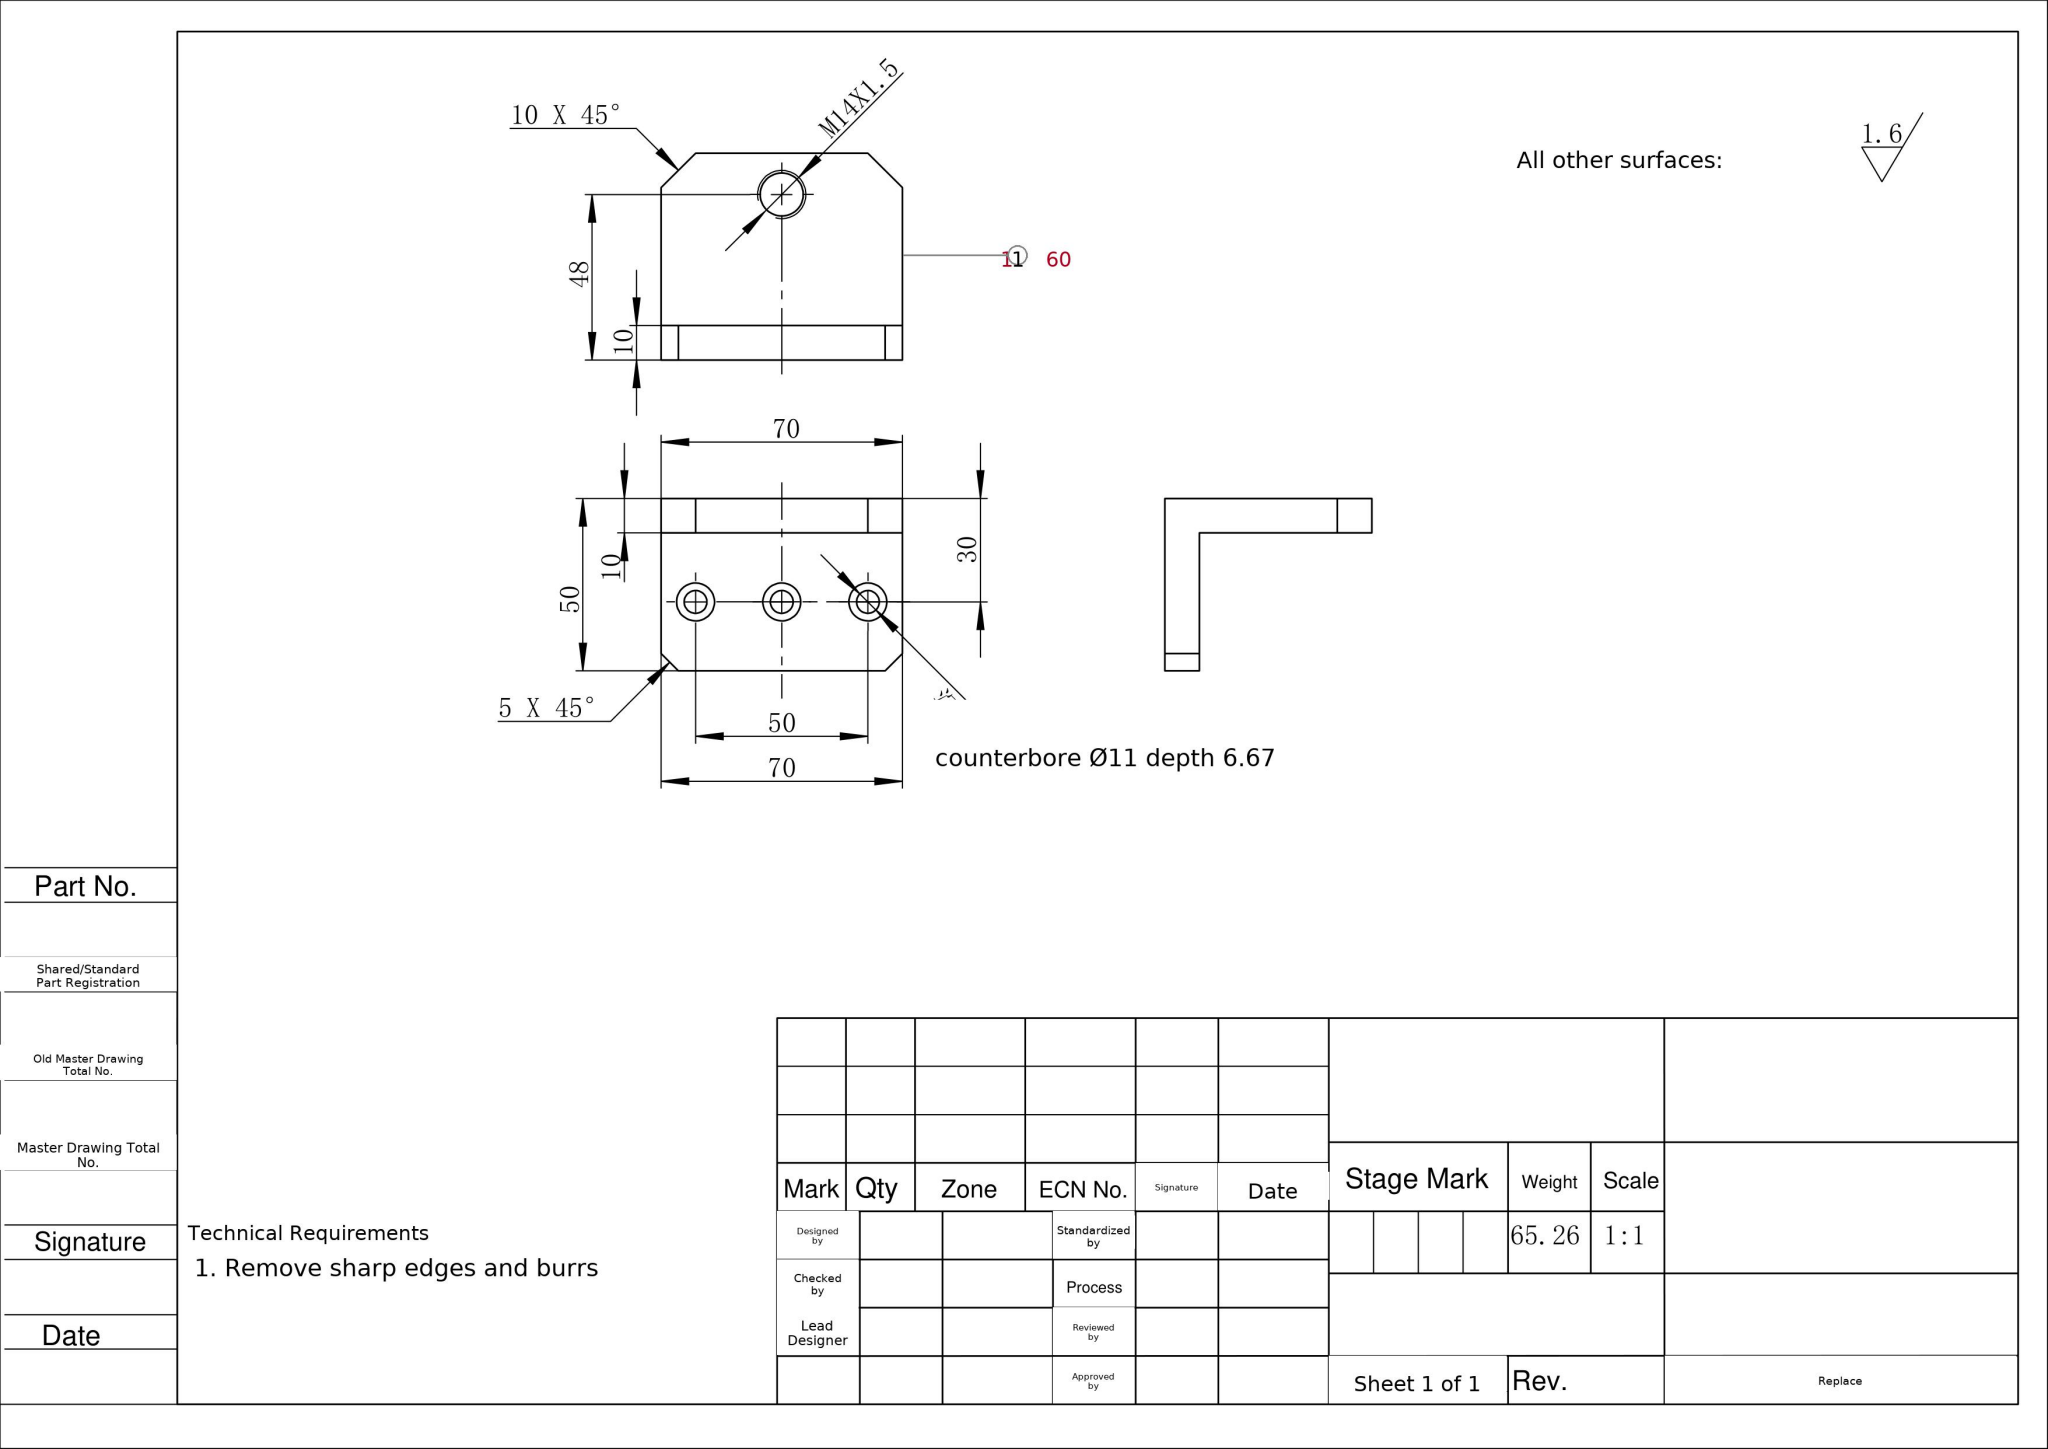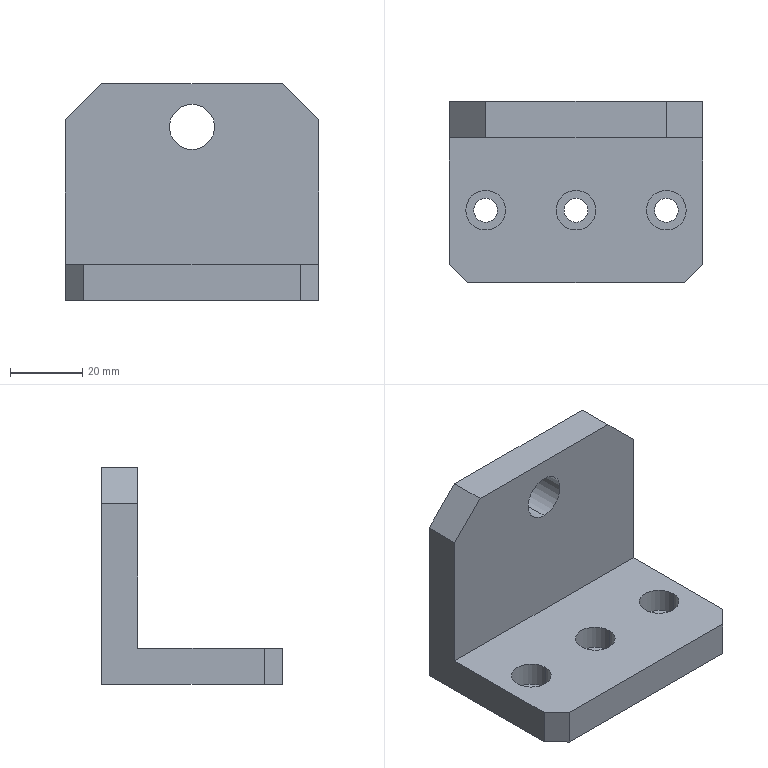Part | SolidWorks | mm | 1 solid | 29 faces | box 70 x 50 x 60 mm | volume 65256 mm3 | plane 15 | cylinder 14 | commonest cylinder face diameters 11 x6 6.6 x6 12.5 x2
build123d program:
from build123d import *

# Parameters (mm, degrees)
SKETCH1_W                                         = 70
SKETCH1_H                                         = 50
BOSS_EXTRUDE1_DEPTH                               = 10
SKETCH2_W                                         = 70
SKETCH2_H                                         = 10
BOSS_EXTRUDE2_DEPTH                               = 50
M14X1_5_TAPPED_HOLE1_D                            = 12.5
CHAMFER1_SIZE                                     = 10
CHAMFER2_SIZE                                     = 5
HOLE_SIZE_ACCORDING_TO_TYPE_1_OF_HEXA_D           = 6.6
HOLE_SIZE_ACCORDING_TO_TYPE_1_OF_HEXA_CBORE_D     = 11
HOLE_SIZE_ACCORDING_TO_TYPE_1_OF_HEXA_CBORE_DEPTH = 6.8


with BuildPart() as part:
    # Sketch1 → Boss-Extrude1 (new body)
    with BuildSketch(Plane.XY):
        with Locations((-1262.738, -1147.6)):
            Rectangle(SKETCH1_W, SKETCH1_H)
    extrude(amount=BOSS_EXTRUDE1_DEPTH)

    # Sketch2 → Boss-Extrude2 (add)
    with BuildSketch(Plane.XY.offset(10)):
        with Locations((-1262.738, -1127.6)):
            Rectangle(SKETCH2_W, SKETCH2_H)
    extrude(amount=BOSS_EXTRUDE2_DEPTH)

    # M14x1.5 Tapped Hole1 (through all)
    with Locations(Plane(origin=(0, -1132.6, 0), x_dir=(-1, 0, 0), z_dir=(0, -1, 0))):
        with Locations((1262.738, -48)):
            Hole(M14X1_5_TAPPED_HOLE1_D / 2)

    # Chamfer1
    chamfer1_edges = [part.edges().sort_by_distance(p)[0] for p in [
        (-1297.738, -1127.6, 60),
        (-1227.738, -1127.6, 60),
    ]]
    chamfer(chamfer1_edges, length=CHAMFER1_SIZE)

    # Chamfer2
    chamfer2_edges = [part.edges().sort_by_distance(p)[0] for p in [
        (-1227.738, -1172.6, 5),
        (-1297.738, -1172.6, 5),
    ]]
    chamfer(chamfer2_edges, length=CHAMFER2_SIZE)

    # Hole Size _ according to_ Type 1 of Hexa (through all)
    with Locations(Plane.XY.offset(10)):
        with Locations((-1287.738, -1152.6), (-1237.738, -1152.6), (-1262.738, -1152.6)):
            CounterBoreHole(HOLE_SIZE_ACCORDING_TO_TYPE_1_OF_HEXA_D / 2, HOLE_SIZE_ACCORDING_TO_TYPE_1_OF_HEXA_CBORE_D / 2, HOLE_SIZE_ACCORDING_TO_TYPE_1_OF_HEXA_CBORE_DEPTH)


solid = part.part
STEP:
#1=CARTESIAN_POINT('',(-1293.238,-1152.6,3.2));
#2=VERTEX_POINT('',#1);
#3=CARTESIAN_POINT('',(-1282.238,-1152.6,3.2));
#4=VERTEX_POINT('',#3);
#5=CARTESIAN_POINT('',(-1287.738,-1152.6,3.2));
#6=DIRECTION('',(0.,0.,1.));
#7=DIRECTION('',(1.,0.,0.));
#8=AXIS2_PLACEMENT_3D('',#5,#6,#7);
#9=CIRCLE('',#8,5.5);
#10=EDGE_CURVE('',#2,#4,#9,.T.);
#11=ORIENTED_EDGE('',*,*,#10,.F.);
#12=CARTESIAN_POINT('',(-1293.238,-1152.6,10.));
#13=VERTEX_POINT('',#12);
#14=CARTESIAN_POINT('',(-1293.238,-1152.6,10.));
#15=DIRECTION('',(0.,0.,1.));
#16=VECTOR('',#15,1000.);
#17=LINE('',#14,#16);
#18=EDGE_CURVE('',#2,#13,#17,.T.);
#19=ORIENTED_EDGE('',*,*,#18,.T.);
#20=CARTESIAN_POINT('',(-1282.238,-1152.6,10.));
#21=VERTEX_POINT('',#20);
#22=CARTESIAN_POINT('',(-1287.738,-1152.6,10.));
#23=DIRECTION('',(0.,0.,1.));
#24=DIRECTION('',(1.,0.,0.));
#25=AXIS2_PLACEMENT_3D('',#22,#23,#24);
#26=CIRCLE('',#25,5.5);
#27=EDGE_CURVE('',#13,#21,#26,.T.);
#28=ORIENTED_EDGE('',*,*,#27,.T.);
#29=CARTESIAN_POINT('',(-1282.238,-1152.6,10.));
#30=DIRECTION('',(0.,0.,1.));
#31=VECTOR('',#30,1000.);
#32=LINE('',#29,#31);
#33=EDGE_CURVE('',#4,#21,#32,.T.);
#34=ORIENTED_EDGE('',*,*,#33,.F.);
#35=EDGE_LOOP('',(#11,#19,#28,#34));
#36=FACE_OUTER_BOUND('',#35,.T.);
#37=CARTESIAN_POINT('',(-1287.738,-1152.6,10.));
#38=DIRECTION('',(0.,0.,1.));
#39=DIRECTION('',(1.,0.,0.));
#40=AXIS2_PLACEMENT_3D('',#37,#38,#39);
#41=CYLINDRICAL_SURFACE('',#40,5.5);
#42=ADVANCED_FACE('',(#36),#41,.F.);
#43=CARTESIAN_POINT('',(-1291.038,-1152.6,0.));
#44=VERTEX_POINT('',#43);
#45=CARTESIAN_POINT('',(-1284.438,-1152.6,0.));
#46=VERTEX_POINT('',#45);
#47=CARTESIAN_POINT('',(-1287.738,-1152.6,0.));
#48=DIRECTION('',(0.,0.,1.));
#49=DIRECTION('',(1.,0.,0.));
#50=AXIS2_PLACEMENT_3D('',#47,#48,#49);
#51=CIRCLE('',#50,3.3);
#52=EDGE_CURVE('',#44,#46,#51,.T.);
#53=ORIENTED_EDGE('',*,*,#52,.F.);
#54=CARTESIAN_POINT('',(-1291.038,-1152.6,3.2));
#55=VERTEX_POINT('',#54);
#56=CARTESIAN_POINT('',(-1291.038,-1152.6,10.));
#57=DIRECTION('',(0.,0.,1.));
#58=VECTOR('',#57,1000.);
#59=LINE('',#56,#58);
#60=EDGE_CURVE('',#44,#55,#59,.T.);
#61=ORIENTED_EDGE('',*,*,#60,.T.);
#62=CARTESIAN_POINT('',(-1284.438,-1152.6,3.2));
#63=VERTEX_POINT('',#62);
#64=CARTESIAN_POINT('',(-1287.738,-1152.6,3.2));
#65=DIRECTION('',(0.,0.,1.));
#66=DIRECTION('',(1.,0.,0.));
#67=AXIS2_PLACEMENT_3D('',#64,#65,#66);
#68=CIRCLE('',#67,3.3);
#69=EDGE_CURVE('',#55,#63,#68,.T.);
#70=ORIENTED_EDGE('',*,*,#69,.T.);
#71=CARTESIAN_POINT('',(-1284.438,-1152.6,10.));
#72=DIRECTION('',(0.,0.,1.));
#73=VECTOR('',#72,1000.);
#74=LINE('',#71,#73);
#75=EDGE_CURVE('',#46,#63,#74,.T.);
#76=ORIENTED_EDGE('',*,*,#75,.F.);
#77=EDGE_LOOP('',(#53,#61,#70,#76));
#78=FACE_OUTER_BOUND('',#77,.T.);
#79=CARTESIAN_POINT('',(-1287.738,-1152.6,10.));
#80=DIRECTION('',(0.,0.,1.));
#81=DIRECTION('',(1.,0.,0.));
#82=AXIS2_PLACEMENT_3D('',#79,#80,#81);
#83=CYLINDRICAL_SURFACE('',#82,3.3);
#84=ADVANCED_FACE('',(#78),#83,.F.);
#85=CARTESIAN_POINT('',(-1243.238,-1152.6,3.2));
#86=VERTEX_POINT('',#85);
#87=CARTESIAN_POINT('',(-1232.238,-1152.6,3.2));
#88=VERTEX_POINT('',#87);
#89=CARTESIAN_POINT('',(-1237.738,-1152.6,3.2));
#90=DIRECTION('',(0.,0.,1.));
#91=DIRECTION('',(1.,0.,0.));
#92=AXIS2_PLACEMENT_3D('',#89,#90,#91);
#93=CIRCLE('',#92,5.5);
#94=EDGE_CURVE('',#86,#88,#93,.T.);
#95=ORIENTED_EDGE('',*,*,#94,.F.);
#96=CARTESIAN_POINT('',(-1243.238,-1152.6,10.));
#97=VERTEX_POINT('',#96);
#98=CARTESIAN_POINT('',(-1243.238,-1152.6,10.));
#99=DIRECTION('',(0.,0.,1.));
#100=VECTOR('',#99,1000.);
#101=LINE('',#98,#100);
#102=EDGE_CURVE('',#86,#97,#101,.T.);
#103=ORIENTED_EDGE('',*,*,#102,.T.);
#104=CARTESIAN_POINT('',(-1232.238,-1152.6,10.));
#105=VERTEX_POINT('',#104);
#106=CARTESIAN_POINT('',(-1237.738,-1152.6,10.));
#107=DIRECTION('',(0.,0.,1.));
#108=DIRECTION('',(1.,0.,0.));
#109=AXIS2_PLACEMENT_3D('',#106,#107,#108);
#110=CIRCLE('',#109,5.5);
#111=EDGE_CURVE('',#97,#105,#110,.T.);
#112=ORIENTED_EDGE('',*,*,#111,.T.);
#113=CARTESIAN_POINT('',(-1232.238,-1152.6,10.));
#114=DIRECTION('',(0.,0.,1.));
#115=VECTOR('',#114,1000.);
#116=LINE('',#113,#115);
#117=EDGE_CURVE('',#88,#105,#116,.T.);
#118=ORIENTED_EDGE('',*,*,#117,.F.);
#119=EDGE_LOOP('',(#95,#103,#112,#118));
#120=FACE_OUTER_BOUND('',#119,.T.);
#121=CARTESIAN_POINT('',(-1237.738,-1152.6,10.));
#122=DIRECTION('',(0.,0.,1.));
#123=DIRECTION('',(1.,0.,0.));
#124=AXIS2_PLACEMENT_3D('',#121,#122,#123);
#125=CYLINDRICAL_SURFACE('',#124,5.5);
#126=ADVANCED_FACE('',(#120),#125,.F.);
#127=CARTESIAN_POINT('',(-1241.038,-1152.6,0.));
#128=VERTEX_POINT('',#127);
#129=CARTESIAN_POINT('',(-1234.438,-1152.6,0.));
#130=VERTEX_POINT('',#129);
#131=CARTESIAN_POINT('',(-1237.738,-1152.6,0.));
#132=DIRECTION('',(0.,0.,1.));
#133=DIRECTION('',(1.,0.,0.));
#134=AXIS2_PLACEMENT_3D('',#131,#132,#133);
#135=CIRCLE('',#134,3.3);
#136=EDGE_CURVE('',#128,#130,#135,.T.);
#137=ORIENTED_EDGE('',*,*,#136,.F.);
#138=CARTESIAN_POINT('',(-1241.038,-1152.6,3.2));
#139=VERTEX_POINT('',#138);
#140=CARTESIAN_POINT('',(-1241.038,-1152.6,10.));
#141=DIRECTION('',(0.,0.,1.));
#142=VECTOR('',#141,1000.);
#143=LINE('',#140,#142);
#144=EDGE_CURVE('',#128,#139,#143,.T.);
#145=ORIENTED_EDGE('',*,*,#144,.T.);
#146=CARTESIAN_POINT('',(-1234.438,-1152.6,3.2));
#147=VERTEX_POINT('',#146);
#148=CARTESIAN_POINT('',(-1237.738,-1152.6,3.2));
#149=DIRECTION('',(0.,0.,1.));
#150=DIRECTION('',(1.,0.,0.));
#151=AXIS2_PLACEMENT_3D('',#148,#149,#150);
#152=CIRCLE('',#151,3.3);
#153=EDGE_CURVE('',#139,#147,#152,.T.);
#154=ORIENTED_EDGE('',*,*,#153,.T.);
#155=CARTESIAN_POINT('',(-1234.438,-1152.6,10.));
#156=DIRECTION('',(0.,0.,1.));
#157=VECTOR('',#156,1000.);
#158=LINE('',#155,#157);
#159=EDGE_CURVE('',#130,#147,#158,.T.);
#160=ORIENTED_EDGE('',*,*,#159,.F.);
#161=EDGE_LOOP('',(#137,#145,#154,#160));
#162=FACE_OUTER_BOUND('',#161,.T.);
#163=CARTESIAN_POINT('',(-1237.738,-1152.6,10.));
#164=DIRECTION('',(0.,0.,1.));
#165=DIRECTION('',(1.,0.,0.));
#166=AXIS2_PLACEMENT_3D('',#163,#164,#165);
#167=CYLINDRICAL_SURFACE('',#166,3.3);
#168=ADVANCED_FACE('',(#162),#167,.F.);
#169=CARTESIAN_POINT('',(-1268.238,-1152.6,3.2));
#170=VERTEX_POINT('',#169);
#171=CARTESIAN_POINT('',(-1257.238,-1152.6,3.2));
#172=VERTEX_POINT('',#171);
#173=CARTESIAN_POINT('',(-1262.738,-1152.6,3.2));
#174=DIRECTION('',(0.,0.,1.));
#175=DIRECTION('',(1.,0.,0.));
#176=AXIS2_PLACEMENT_3D('',#173,#174,#175);
#177=CIRCLE('',#176,5.5);
#178=EDGE_CURVE('',#170,#172,#177,.T.);
#179=ORIENTED_EDGE('',*,*,#178,.F.);
#180=CARTESIAN_POINT('',(-1268.238,-1152.6,10.));
#181=VERTEX_POINT('',#180);
#182=CARTESIAN_POINT('',(-1268.238,-1152.6,10.));
#183=DIRECTION('',(0.,0.,1.));
#184=VECTOR('',#183,1000.);
#185=LINE('',#182,#184);
#186=EDGE_CURVE('',#170,#181,#185,.T.);
#187=ORIENTED_EDGE('',*,*,#186,.T.);
#188=CARTESIAN_POINT('',(-1257.238,-1152.6,10.));
#189=VERTEX_POINT('',#188);
#190=CARTESIAN_POINT('',(-1262.738,-1152.6,10.));
#191=DIRECTION('',(0.,0.,1.));
#192=DIRECTION('',(1.,0.,0.));
#193=AXIS2_PLACEMENT_3D('',#190,#191,#192);
#194=CIRCLE('',#193,5.5);
#195=EDGE_CURVE('',#181,#189,#194,.T.);
#196=ORIENTED_EDGE('',*,*,#195,.T.);
#197=CARTESIAN_POINT('',(-1257.238,-1152.6,10.));
#198=DIRECTION('',(0.,0.,1.));
#199=VECTOR('',#198,1000.);
#200=LINE('',#197,#199);
#201=EDGE_CURVE('',#172,#189,#200,.T.);
#202=ORIENTED_EDGE('',*,*,#201,.F.);
#203=EDGE_LOOP('',(#179,#187,#196,#202));
#204=FACE_OUTER_BOUND('',#203,.T.);
#205=CARTESIAN_POINT('',(-1262.738,-1152.6,10.));
#206=DIRECTION('',(0.,0.,1.));
#207=DIRECTION('',(1.,0.,0.));
#208=AXIS2_PLACEMENT_3D('',#205,#206,#207);
#209=CYLINDRICAL_SURFACE('',#208,5.5);
#210=ADVANCED_FACE('',(#204),#209,.F.);
#211=CARTESIAN_POINT('',(-1266.038,-1152.6,0.));
#212=VERTEX_POINT('',#211);
#213=CARTESIAN_POINT('',(-1259.438,-1152.6,0.));
#214=VERTEX_POINT('',#213);
#215=CARTESIAN_POINT('',(-1262.738,-1152.6,0.));
#216=DIRECTION('',(0.,0.,1.));
#217=DIRECTION('',(1.,0.,0.));
#218=AXIS2_PLACEMENT_3D('',#215,#216,#217);
#219=CIRCLE('',#218,3.3);
#220=EDGE_CURVE('',#212,#214,#219,.T.);
#221=ORIENTED_EDGE('',*,*,#220,.F.);
#222=CARTESIAN_POINT('',(-1266.038,-1152.6,3.2));
#223=VERTEX_POINT('',#222);
#224=CARTESIAN_POINT('',(-1266.038,-1152.6,10.));
#225=DIRECTION('',(0.,0.,1.));
#226=VECTOR('',#225,1000.);
#227=LINE('',#224,#226);
#228=EDGE_CURVE('',#212,#223,#227,.T.);
#229=ORIENTED_EDGE('',*,*,#228,.T.);
#230=CARTESIAN_POINT('',(-1259.438,-1152.6,3.2));
#231=VERTEX_POINT('',#230);
#232=CARTESIAN_POINT('',(-1262.738,-1152.6,3.2));
#233=DIRECTION('',(0.,0.,1.));
#234=DIRECTION('',(1.,0.,0.));
#235=AXIS2_PLACEMENT_3D('',#232,#233,#234);
#236=CIRCLE('',#235,3.3);
#237=EDGE_CURVE('',#223,#231,#236,.T.);
#238=ORIENTED_EDGE('',*,*,#237,.T.);
#239=CARTESIAN_POINT('',(-1259.438,-1152.6,10.));
#240=DIRECTION('',(0.,0.,1.));
#241=VECTOR('',#240,1000.);
#242=LINE('',#239,#241);
#243=EDGE_CURVE('',#214,#231,#242,.T.);
#244=ORIENTED_EDGE('',*,*,#243,.F.);
#245=EDGE_LOOP('',(#221,#229,#238,#244));
#246=FACE_OUTER_BOUND('',#245,.T.);
#247=CARTESIAN_POINT('',(-1262.738,-1152.6,10.));
#248=DIRECTION('',(0.,0.,1.));
#249=DIRECTION('',(1.,0.,0.));
#250=AXIS2_PLACEMENT_3D('',#247,#248,#249);
#251=CYLINDRICAL_SURFACE('',#250,3.3);
#252=ADVANCED_FACE('',(#246),#251,.F.);
#253=CARTESIAN_POINT('',(-1262.738,-1122.6,54.25));
#254=VERTEX_POINT('',#253);
#255=CARTESIAN_POINT('',(-1262.738,-1122.6,41.75));
#256=VERTEX_POINT('',#255);
#257=CARTESIAN_POINT('',(-1262.738,-1122.6,48.));
#258=DIRECTION('',(0.,-1.,0.));
#259=DIRECTION('',(0.,0.,-1.));
#260=AXIS2_PLACEMENT_3D('',#257,#258,#259);
#261=CIRCLE('',#260,6.25);
#262=EDGE_CURVE('',#254,#256,#261,.T.);
#263=ORIENTED_EDGE('',*,*,#262,.F.);
#264=CARTESIAN_POINT('',(-1262.738,-1132.6,54.25));
#265=VERTEX_POINT('',#264);
#266=CARTESIAN_POINT('',(-1262.738,-1132.6,54.25));
#267=DIRECTION('',(0.,-1.,0.));
#268=VECTOR('',#267,1000.);
#269=LINE('',#266,#268);
#270=EDGE_CURVE('',#254,#265,#269,.T.);
#271=ORIENTED_EDGE('',*,*,#270,.T.);
#272=CARTESIAN_POINT('',(-1262.738,-1132.6,41.75));
#273=VERTEX_POINT('',#272);
#274=CARTESIAN_POINT('',(-1262.738,-1132.6,48.));
#275=DIRECTION('',(0.,-1.,0.));
#276=DIRECTION('',(0.,0.,-1.));
#277=AXIS2_PLACEMENT_3D('',#274,#275,#276);
#278=CIRCLE('',#277,6.25);
#279=EDGE_CURVE('',#265,#273,#278,.T.);
#280=ORIENTED_EDGE('',*,*,#279,.T.);
#281=CARTESIAN_POINT('',(-1262.738,-1132.6,41.75));
#282=DIRECTION('',(0.,-1.,0.));
#283=VECTOR('',#282,1000.);
#284=LINE('',#281,#283);
#285=EDGE_CURVE('',#256,#273,#284,.T.);
#286=ORIENTED_EDGE('',*,*,#285,.F.);
#287=EDGE_LOOP('',(#263,#271,#280,#286));
#288=FACE_OUTER_BOUND('',#287,.T.);
#289=CARTESIAN_POINT('',(-1262.738,-1132.6,48.));
#290=DIRECTION('',(0.,-1.,0.));
#291=DIRECTION('',(0.,0.,-1.));
#292=AXIS2_PLACEMENT_3D('',#289,#290,#291);
#293=CYLINDRICAL_SURFACE('',#292,6.25);
#294=ADVANCED_FACE('',(#288),#293,.F.);
#295=CARTESIAN_POINT('',(-1297.738,-1122.6,0.));
#296=VERTEX_POINT('',#295);
#297=CARTESIAN_POINT('',(-1297.738,-1167.6,0.));
#298=VERTEX_POINT('',#297);
#299=CARTESIAN_POINT('',(-1297.738,-1122.6,0.));
#300=DIRECTION('',(0.,-1.,0.));
#301=VECTOR('',#300,1000.);
#302=LINE('',#299,#301);
#303=EDGE_CURVE('',#296,#298,#302,.T.);
#304=ORIENTED_EDGE('',*,*,#303,.T.);
#305=CARTESIAN_POINT('',(-1297.738,-1167.6,10.));
#306=VERTEX_POINT('',#305);
#307=CARTESIAN_POINT('',(-1297.738,-1167.6,10.));
#308=DIRECTION('',(0.,0.,1.));
#309=VECTOR('',#308,1000.);
#310=LINE('',#307,#309);
#311=EDGE_CURVE('',#298,#306,#310,.T.);
#312=ORIENTED_EDGE('',*,*,#311,.T.);
#313=CARTESIAN_POINT('',(-1297.738,-1132.6,10.));
#314=VERTEX_POINT('',#313);
#315=CARTESIAN_POINT('',(-1297.738,-1122.6,10.));
#316=DIRECTION('',(0.,-1.,0.));
#317=VECTOR('',#316,1000.);
#318=LINE('',#315,#317);
#319=EDGE_CURVE('',#314,#306,#318,.T.);
#320=ORIENTED_EDGE('',*,*,#319,.F.);
#321=CARTESIAN_POINT('',(-1297.738,-1132.6,50.));
#322=VERTEX_POINT('',#321);
#323=CARTESIAN_POINT('',(-1297.738,-1132.6,60.));
#324=DIRECTION('',(0.,0.,-1.));
#325=VECTOR('',#324,1000.);
#326=LINE('',#323,#325);
#327=EDGE_CURVE('',#322,#314,#326,.T.);
#328=ORIENTED_EDGE('',*,*,#327,.F.);
#329=CARTESIAN_POINT('',(-1297.738,-1122.6,50.));
#330=VERTEX_POINT('',#329);
#331=CARTESIAN_POINT('',(-1297.738,-1122.6,50.));
#332=DIRECTION('',(-0.,1.,0.));
#333=VECTOR('',#332,1000.);
#334=LINE('',#331,#333);
#335=EDGE_CURVE('',#322,#330,#334,.T.);
#336=ORIENTED_EDGE('',*,*,#335,.T.);
#337=CARTESIAN_POINT('',(-1297.738,-1122.6,10.));
#338=DIRECTION('',(0.,0.,-1.));
#339=VECTOR('',#338,1000.);
#340=LINE('',#337,#339);
#341=EDGE_CURVE('',#330,#296,#340,.T.);
#342=ORIENTED_EDGE('',*,*,#341,.T.);
#343=EDGE_LOOP('',(#304,#312,#320,#328,#336,#342));
#344=FACE_OUTER_BOUND('',#343,.T.);
#345=CARTESIAN_POINT('',(-1297.738,-1122.6,10.));
#346=DIRECTION('',(1.,0.,0.));
#347=DIRECTION('',(-0.,1.,0.));
#348=AXIS2_PLACEMENT_3D('',#345,#346,#347);
#349=PLANE('',#348);
#350=ADVANCED_FACE('',(#344),#349,.F.);
#351=CARTESIAN_POINT('',(-1292.738,-1172.6,0.));
#352=VERTEX_POINT('',#351);
#353=CARTESIAN_POINT('',(-1232.738,-1172.6,0.));
#354=VERTEX_POINT('',#353);
#355=CARTESIAN_POINT('',(-1297.738,-1172.6,0.));
#356=DIRECTION('',(1.,0.,0.));
#357=VECTOR('',#356,1000.);
#358=LINE('',#355,#357);
#359=EDGE_CURVE('',#352,#354,#358,.T.);
#360=ORIENTED_EDGE('',*,*,#359,.T.);
#361=CARTESIAN_POINT('',(-1232.738,-1172.6,10.));
#362=VERTEX_POINT('',#361);
#363=CARTESIAN_POINT('',(-1232.738,-1172.6,10.));
#364=DIRECTION('',(0.,0.,1.));
#365=VECTOR('',#364,1000.);
#366=LINE('',#363,#365);
#367=EDGE_CURVE('',#354,#362,#366,.T.);
#368=ORIENTED_EDGE('',*,*,#367,.T.);
#369=CARTESIAN_POINT('',(-1292.738,-1172.6,10.));
#370=VERTEX_POINT('',#369);
#371=CARTESIAN_POINT('',(-1297.738,-1172.6,10.));
#372=DIRECTION('',(1.,0.,0.));
#373=VECTOR('',#372,1000.);
#374=LINE('',#371,#373);
#375=EDGE_CURVE('',#370,#362,#374,.T.);
#376=ORIENTED_EDGE('',*,*,#375,.F.);
#377=CARTESIAN_POINT('',(-1292.738,-1172.6,10.));
#378=DIRECTION('',(0.,0.,-1.));
#379=VECTOR('',#378,1000.);
#380=LINE('',#377,#379);
#381=EDGE_CURVE('',#370,#352,#380,.T.);
#382=ORIENTED_EDGE('',*,*,#381,.T.);
#383=EDGE_LOOP('',(#360,#368,#376,#382));
#384=FACE_OUTER_BOUND('',#383,.T.);
#385=CARTESIAN_POINT('',(-1297.738,-1172.6,10.));
#386=DIRECTION('',(0.,1.,0.));
#387=DIRECTION('',(0.,0.,1.));
#388=AXIS2_PLACEMENT_3D('',#385,#386,#387);
#389=PLANE('',#388);
#390=ADVANCED_FACE('',(#384),#389,.F.);
#391=CARTESIAN_POINT('',(-1227.738,-1167.6,10.));
#392=VERTEX_POINT('',#391);
#393=CARTESIAN_POINT('',(-1227.738,-1132.6,10.));
#394=VERTEX_POINT('',#393);
#395=CARTESIAN_POINT('',(-1227.738,-1122.6,10.));
#396=DIRECTION('',(0.,1.,0.));
#397=VECTOR('',#396,1000.);
#398=LINE('',#395,#397);
#399=EDGE_CURVE('',#392,#394,#398,.T.);
#400=ORIENTED_EDGE('',*,*,#399,.F.);
#401=CARTESIAN_POINT('',(-1227.738,-1167.6,0.));
#402=VERTEX_POINT('',#401);
#403=CARTESIAN_POINT('',(-1227.738,-1167.6,10.));
#404=DIRECTION('',(0.,0.,-1.));
#405=VECTOR('',#404,1000.);
#406=LINE('',#403,#405);
#407=EDGE_CURVE('',#392,#402,#406,.T.);
#408=ORIENTED_EDGE('',*,*,#407,.T.);
#409=CARTESIAN_POINT('',(-1227.738,-1122.6,0.));
#410=VERTEX_POINT('',#409);
#411=CARTESIAN_POINT('',(-1227.738,-1122.6,0.));
#412=DIRECTION('',(0.,1.,0.));
#413=VECTOR('',#412,1000.);
#414=LINE('',#411,#413);
#415=EDGE_CURVE('',#402,#410,#414,.T.);
#416=ORIENTED_EDGE('',*,*,#415,.T.);
#417=CARTESIAN_POINT('',(-1227.738,-1122.6,50.));
#418=VERTEX_POINT('',#417);
#419=CARTESIAN_POINT('',(-1227.738,-1122.6,10.));
#420=DIRECTION('',(0.,0.,-1.));
#421=VECTOR('',#420,1000.);
#422=LINE('',#419,#421);
#423=EDGE_CURVE('',#418,#410,#422,.T.);
#424=ORIENTED_EDGE('',*,*,#423,.F.);
#425=CARTESIAN_POINT('',(-1227.738,-1132.6,50.));
#426=VERTEX_POINT('',#425);
#427=CARTESIAN_POINT('',(-1227.738,-1132.6,50.));
#428=DIRECTION('',(-0.,-1.,0.));
#429=VECTOR('',#428,1000.);
#430=LINE('',#427,#429);
#431=EDGE_CURVE('',#418,#426,#430,.T.);
#432=ORIENTED_EDGE('',*,*,#431,.T.);
#433=CARTESIAN_POINT('',(-1227.738,-1132.6,60.));
#434=DIRECTION('',(0.,0.,-1.));
#435=VECTOR('',#434,1000.);
#436=LINE('',#433,#435);
#437=EDGE_CURVE('',#426,#394,#436,.T.);
#438=ORIENTED_EDGE('',*,*,#437,.T.);
#439=EDGE_LOOP('',(#400,#408,#416,#424,#432,#438));
#440=FACE_OUTER_BOUND('',#439,.T.);
#441=CARTESIAN_POINT('',(-1227.738,-1122.6,10.));
#442=DIRECTION('',(-1.,0.,0.));
#443=DIRECTION('',(-0.,-1.,0.));
#444=AXIS2_PLACEMENT_3D('',#441,#442,#443);
#445=PLANE('',#444);
#446=ADVANCED_FACE('',(#440),#445,.F.);
#447=CARTESIAN_POINT('',(-1262.738,-1122.6,48.));
#448=DIRECTION('',(0.,-1.,0.));
#449=DIRECTION('',(0.,0.,-1.));
#450=AXIS2_PLACEMENT_3D('',#447,#448,#449);
#451=CIRCLE('',#450,6.25);
#452=EDGE_CURVE('',#256,#254,#451,.T.);
#453=ORIENTED_EDGE('',*,*,#452,.T.);
#454=ORIENTED_EDGE('',*,*,#262,.T.);
#455=EDGE_LOOP('',(#453,#454));
#456=FACE_BOUND('',#455,.T.);
#457=CARTESIAN_POINT('',(-1237.738,-1122.6,60.));
#458=VERTEX_POINT('',#457);
#459=CARTESIAN_POINT('',(-1287.738,-1122.6,60.));
#460=VERTEX_POINT('',#459);
#461=CARTESIAN_POINT('',(-1297.738,-1122.6,60.));
#462=DIRECTION('',(-1.,0.,0.));
#463=VECTOR('',#462,1000.);
#464=LINE('',#461,#463);
#465=EDGE_CURVE('',#458,#460,#464,.T.);
#466=ORIENTED_EDGE('',*,*,#465,.F.);
#467=CARTESIAN_POINT('',(-1237.738,-1122.6,60.));
#468=DIRECTION('',(0.7071,0.,-0.7071));
#469=VECTOR('',#468,1000.);
#470=LINE('',#467,#469);
#471=EDGE_CURVE('',#458,#418,#470,.T.);
#472=ORIENTED_EDGE('',*,*,#471,.T.);
#473=ORIENTED_EDGE('',*,*,#423,.T.);
#474=CARTESIAN_POINT('',(-1297.738,-1122.6,0.));
#475=DIRECTION('',(-1.,0.,0.));
#476=VECTOR('',#475,1000.);
#477=LINE('',#474,#476);
#478=EDGE_CURVE('',#410,#296,#477,.T.);
#479=ORIENTED_EDGE('',*,*,#478,.T.);
#480=ORIENTED_EDGE('',*,*,#341,.F.);
#481=CARTESIAN_POINT('',(-1287.738,-1122.6,60.));
#482=DIRECTION('',(0.7071,0.,0.7071));
#483=VECTOR('',#482,1000.);
#484=LINE('',#481,#483);
#485=EDGE_CURVE('',#330,#460,#484,.T.);
#486=ORIENTED_EDGE('',*,*,#485,.T.);
#487=EDGE_LOOP('',(#466,#472,#473,#479,#480,#486));
#488=FACE_OUTER_BOUND('',#487,.T.);
#489=CARTESIAN_POINT('',(-1297.738,-1122.6,10.));
#490=DIRECTION('',(0.,-1.,0.));
#491=DIRECTION('',(0.,0.,-1.));
#492=AXIS2_PLACEMENT_3D('',#489,#490,#491);
#493=PLANE('',#492);
#494=ADVANCED_FACE('',(#456,#488),#493,.F.);
#495=CARTESIAN_POINT('',(-1287.738,-1152.6,10.));
#496=DIRECTION('',(0.,0.,1.));
#497=DIRECTION('',(1.,0.,0.));
#498=AXIS2_PLACEMENT_3D('',#495,#496,#497);
#499=CIRCLE('',#498,5.5);
#500=EDGE_CURVE('',#21,#13,#499,.T.);
#501=ORIENTED_EDGE('',*,*,#500,.F.);
#502=ORIENTED_EDGE('',*,*,#27,.F.);
#503=EDGE_LOOP('',(#501,#502));
#504=FACE_BOUND('',#503,.T.);
#505=CARTESIAN_POINT('',(-1237.738,-1152.6,10.));
#506=DIRECTION('',(0.,0.,1.));
#507=DIRECTION('',(1.,0.,0.));
#508=AXIS2_PLACEMENT_3D('',#505,#506,#507);
#509=CIRCLE('',#508,5.5);
#510=EDGE_CURVE('',#105,#97,#509,.T.);
#511=ORIENTED_EDGE('',*,*,#510,.F.);
#512=ORIENTED_EDGE('',*,*,#111,.F.);
#513=EDGE_LOOP('',(#511,#512));
#514=FACE_BOUND('',#513,.T.);
#515=CARTESIAN_POINT('',(-1262.738,-1152.6,10.));
#516=DIRECTION('',(0.,0.,1.));
#517=DIRECTION('',(1.,0.,0.));
#518=AXIS2_PLACEMENT_3D('',#515,#516,#517);
#519=CIRCLE('',#518,5.5);
#520=EDGE_CURVE('',#189,#181,#519,.T.);
#521=ORIENTED_EDGE('',*,*,#520,.F.);
#522=ORIENTED_EDGE('',*,*,#195,.F.);
#523=EDGE_LOOP('',(#521,#522));
#524=FACE_BOUND('',#523,.T.);
#525=ORIENTED_EDGE('',*,*,#375,.T.);
#526=CARTESIAN_POINT('',(-30.069,30.069,10.));
#527=DIRECTION('',(0.7071,0.7071,0.));
#528=VECTOR('',#527,1000.);
#529=LINE('',#526,#528);
#530=EDGE_CURVE('',#362,#392,#529,.T.);
#531=ORIENTED_EDGE('',*,*,#530,.T.);
#532=ORIENTED_EDGE('',*,*,#399,.T.);
#533=CARTESIAN_POINT('',(-1297.738,-1132.6,10.));
#534=DIRECTION('',(1.,0.,0.));
#535=VECTOR('',#534,1000.);
#536=LINE('',#533,#535);
#537=EDGE_CURVE('',#314,#394,#536,.T.);
#538=ORIENTED_EDGE('',*,*,#537,.F.);
#539=ORIENTED_EDGE('',*,*,#319,.T.);
#540=CARTESIAN_POINT('',(-1232.669,-1232.669,10.));
#541=DIRECTION('',(0.7071,-0.7071,0.));
#542=VECTOR('',#541,1000.);
#543=LINE('',#540,#542);
#544=EDGE_CURVE('',#306,#370,#543,.T.);
#545=ORIENTED_EDGE('',*,*,#544,.T.);
#546=EDGE_LOOP('',(#525,#531,#532,#538,#539,#545));
#547=FACE_OUTER_BOUND('',#546,.T.);
#548=CARTESIAN_POINT('',(0.,0.,10.));
#549=DIRECTION('',(0.,0.,1.));
#550=DIRECTION('',(1.,0.,0.));
#551=AXIS2_PLACEMENT_3D('',#548,#549,#550);
#552=PLANE('',#551);
#553=ADVANCED_FACE('',(#504,#514,#524,#547),#552,.T.);
#554=CARTESIAN_POINT('',(-1287.738,-1152.6,0.));
#555=DIRECTION('',(0.,0.,1.));
#556=DIRECTION('',(1.,0.,0.));
#557=AXIS2_PLACEMENT_3D('',#554,#555,#556);
#558=CIRCLE('',#557,3.3);
#559=EDGE_CURVE('',#46,#44,#558,.T.);
#560=ORIENTED_EDGE('',*,*,#559,.T.);
#561=ORIENTED_EDGE('',*,*,#52,.T.);
#562=EDGE_LOOP('',(#560,#561));
#563=FACE_BOUND('',#562,.T.);
#564=CARTESIAN_POINT('',(-1237.738,-1152.6,0.));
#565=DIRECTION('',(0.,0.,1.));
#566=DIRECTION('',(1.,0.,0.));
#567=AXIS2_PLACEMENT_3D('',#564,#565,#566);
#568=CIRCLE('',#567,3.3);
#569=EDGE_CURVE('',#130,#128,#568,.T.);
#570=ORIENTED_EDGE('',*,*,#569,.T.);
#571=ORIENTED_EDGE('',*,*,#136,.T.);
#572=EDGE_LOOP('',(#570,#571));
#573=FACE_BOUND('',#572,.T.);
#574=CARTESIAN_POINT('',(-1262.738,-1152.6,0.));
#575=DIRECTION('',(0.,0.,1.));
#576=DIRECTION('',(1.,0.,0.));
#577=AXIS2_PLACEMENT_3D('',#574,#575,#576);
#578=CIRCLE('',#577,3.3);
#579=EDGE_CURVE('',#214,#212,#578,.T.);
#580=ORIENTED_EDGE('',*,*,#579,.T.);
#581=ORIENTED_EDGE('',*,*,#220,.T.);
#582=EDGE_LOOP('',(#580,#581));
#583=FACE_BOUND('',#582,.T.);
#584=ORIENTED_EDGE('',*,*,#415,.F.);
#585=CARTESIAN_POINT('',(-1227.738,-1167.6,0.));
#586=DIRECTION('',(-0.7071,-0.7071,0.));
#587=VECTOR('',#586,1000.);
#588=LINE('',#585,#587);
#589=EDGE_CURVE('',#402,#354,#588,.T.);
#590=ORIENTED_EDGE('',*,*,#589,.T.);
#591=ORIENTED_EDGE('',*,*,#359,.F.);
#592=CARTESIAN_POINT('',(-1292.738,-1172.6,0.));
#593=DIRECTION('',(-0.7071,0.7071,0.));
#594=VECTOR('',#593,1000.);
#595=LINE('',#592,#594);
#596=EDGE_CURVE('',#352,#298,#595,.T.);
#597=ORIENTED_EDGE('',*,*,#596,.T.);
#598=ORIENTED_EDGE('',*,*,#303,.F.);
#599=ORIENTED_EDGE('',*,*,#478,.F.);
#600=EDGE_LOOP('',(#584,#590,#591,#597,#598,#599));
#601=FACE_OUTER_BOUND('',#600,.T.);
#602=CARTESIAN_POINT('',(0.,0.,0.));
#603=DIRECTION('',(0.,0.,1.));
#604=DIRECTION('',(1.,0.,0.));
#605=AXIS2_PLACEMENT_3D('',#602,#603,#604);
#606=PLANE('',#605);
#607=ADVANCED_FACE('',(#563,#573,#583,#601),#606,.F.);
#608=CARTESIAN_POINT('',(-1262.738,-1132.6,48.));
#609=DIRECTION('',(0.,-1.,0.));
#610=DIRECTION('',(0.,0.,-1.));
#611=AXIS2_PLACEMENT_3D('',#608,#609,#610);
#612=CIRCLE('',#611,6.25);
#613=EDGE_CURVE('',#273,#265,#612,.T.);
#614=ORIENTED_EDGE('',*,*,#613,.F.);
#615=ORIENTED_EDGE('',*,*,#279,.F.);
#616=EDGE_LOOP('',(#614,#615));
#617=FACE_BOUND('',#616,.T.);
#618=ORIENTED_EDGE('',*,*,#437,.F.);
#619=CARTESIAN_POINT('',(-1237.738,-1132.6,60.));
#620=VERTEX_POINT('',#619);
#621=CARTESIAN_POINT('',(-1237.738,-1132.6,60.));
#622=DIRECTION('',(-0.7071,0.,0.7071));
#623=VECTOR('',#622,1000.);
#624=LINE('',#621,#623);
#625=EDGE_CURVE('',#426,#620,#624,.T.);
#626=ORIENTED_EDGE('',*,*,#625,.T.);
#627=CARTESIAN_POINT('',(-1287.738,-1132.6,60.));
#628=VERTEX_POINT('',#627);
#629=CARTESIAN_POINT('',(-1297.738,-1132.6,60.));
#630=DIRECTION('',(1.,0.,0.));
#631=VECTOR('',#630,1000.);
#632=LINE('',#629,#631);
#633=EDGE_CURVE('',#628,#620,#632,.T.);
#634=ORIENTED_EDGE('',*,*,#633,.F.);
#635=CARTESIAN_POINT('',(-1287.738,-1132.6,60.));
#636=DIRECTION('',(-0.7071,0.,-0.7071));
#637=VECTOR('',#636,1000.);
#638=LINE('',#635,#637);
#639=EDGE_CURVE('',#628,#322,#638,.T.);
#640=ORIENTED_EDGE('',*,*,#639,.T.);
#641=ORIENTED_EDGE('',*,*,#327,.T.);
#642=ORIENTED_EDGE('',*,*,#537,.T.);
#643=EDGE_LOOP('',(#618,#626,#634,#640,#641,#642));
#644=FACE_OUTER_BOUND('',#643,.T.);
#645=CARTESIAN_POINT('',(-1297.738,-1132.6,60.));
#646=DIRECTION('',(0.,1.,0.));
#647=DIRECTION('',(0.,0.,1.));
#648=AXIS2_PLACEMENT_3D('',#645,#646,#647);
#649=PLANE('',#648);
#650=ADVANCED_FACE('',(#617,#644),#649,.F.);
#651=ORIENTED_EDGE('',*,*,#633,.T.);
#652=CARTESIAN_POINT('',(-1237.738,-1122.6,60.));
#653=DIRECTION('',(0.,1.,0.));
#654=VECTOR('',#653,1000.);
#655=LINE('',#652,#654);
#656=EDGE_CURVE('',#620,#458,#655,.T.);
#657=ORIENTED_EDGE('',*,*,#656,.T.);
#658=ORIENTED_EDGE('',*,*,#465,.T.);
#659=CARTESIAN_POINT('',(-1287.738,-1132.6,60.));
#660=DIRECTION('',(0.,-1.,0.));
#661=VECTOR('',#660,1000.);
#662=LINE('',#659,#661);
#663=EDGE_CURVE('',#460,#628,#662,.T.);
#664=ORIENTED_EDGE('',*,*,#663,.T.);
#665=EDGE_LOOP('',(#651,#657,#658,#664));
#666=FACE_OUTER_BOUND('',#665,.T.);
#667=CARTESIAN_POINT('',(0.,0.,60.));
#668=DIRECTION('',(0.,0.,1.));
#669=DIRECTION('',(1.,0.,0.));
#670=AXIS2_PLACEMENT_3D('',#667,#668,#669);
#671=PLANE('',#670);
#672=ADVANCED_FACE('',(#666),#671,.T.);
#673=ORIENTED_EDGE('',*,*,#270,.F.);
#674=ORIENTED_EDGE('',*,*,#452,.F.);
#675=ORIENTED_EDGE('',*,*,#285,.T.);
#676=ORIENTED_EDGE('',*,*,#613,.T.);
#677=EDGE_LOOP('',(#673,#674,#675,#676));
#678=FACE_OUTER_BOUND('',#677,.T.);
#679=CARTESIAN_POINT('',(-1262.738,-1132.6,48.));
#680=DIRECTION('',(0.,-1.,0.));
#681=DIRECTION('',(0.,0.,-1.));
#682=AXIS2_PLACEMENT_3D('',#679,#680,#681);
#683=CYLINDRICAL_SURFACE('',#682,6.25);
#684=ADVANCED_FACE('',(#678),#683,.F.);
#685=ORIENTED_EDGE('',*,*,#625,.F.);
#686=ORIENTED_EDGE('',*,*,#431,.F.);
#687=ORIENTED_EDGE('',*,*,#471,.F.);
#688=ORIENTED_EDGE('',*,*,#656,.F.);
#689=EDGE_LOOP('',(#685,#686,#687,#688));
#690=FACE_OUTER_BOUND('',#689,.T.);
#691=CARTESIAN_POINT('',(-1237.738,0.,60.));
#692=DIRECTION('',(0.7071,-0.,0.7071));
#693=DIRECTION('',(-0.,-1.,0.));
#694=AXIS2_PLACEMENT_3D('',#691,#692,#693);
#695=PLANE('',#694);
#696=ADVANCED_FACE('',(#690),#695,.T.);
#697=ORIENTED_EDGE('',*,*,#485,.F.);
#698=ORIENTED_EDGE('',*,*,#335,.F.);
#699=ORIENTED_EDGE('',*,*,#639,.F.);
#700=ORIENTED_EDGE('',*,*,#663,.F.);
#701=EDGE_LOOP('',(#697,#698,#699,#700));
#702=FACE_OUTER_BOUND('',#701,.T.);
#703=CARTESIAN_POINT('',(-1287.738,-0.,60.));
#704=DIRECTION('',(-0.7071,-0.,0.7071));
#705=DIRECTION('',(-0.,1.,0.));
#706=AXIS2_PLACEMENT_3D('',#703,#704,#705);
#707=PLANE('',#706);
#708=ADVANCED_FACE('',(#702),#707,.T.);
#709=ORIENTED_EDGE('',*,*,#530,.F.);
#710=ORIENTED_EDGE('',*,*,#367,.F.);
#711=ORIENTED_EDGE('',*,*,#589,.F.);
#712=ORIENTED_EDGE('',*,*,#407,.F.);
#713=EDGE_LOOP('',(#709,#710,#711,#712));
#714=FACE_OUTER_BOUND('',#713,.T.);
#715=CARTESIAN_POINT('',(-1227.738,-1167.6,10.));
#716=DIRECTION('',(-0.7071,0.7071,0.));
#717=DIRECTION('',(0.,0.,-1.));
#718=AXIS2_PLACEMENT_3D('',#715,#716,#717);
#719=PLANE('',#718);
#720=ADVANCED_FACE('',(#714),#719,.F.);
#721=ORIENTED_EDGE('',*,*,#544,.F.);
#722=ORIENTED_EDGE('',*,*,#311,.F.);
#723=ORIENTED_EDGE('',*,*,#596,.F.);
#724=ORIENTED_EDGE('',*,*,#381,.F.);
#725=EDGE_LOOP('',(#721,#722,#723,#724));
#726=FACE_OUTER_BOUND('',#725,.T.);
#727=CARTESIAN_POINT('',(-1292.738,-1172.6,10.));
#728=DIRECTION('',(0.7071,0.7071,0.));
#729=DIRECTION('',(0.,0.,-1.));
#730=AXIS2_PLACEMENT_3D('',#727,#728,#729);
#731=PLANE('',#730);
#732=ADVANCED_FACE('',(#726),#731,.F.);
#733=ORIENTED_EDGE('',*,*,#228,.F.);
#734=ORIENTED_EDGE('',*,*,#579,.F.);
#735=ORIENTED_EDGE('',*,*,#243,.T.);
#736=CARTESIAN_POINT('',(-1262.738,-1152.6,3.2));
#737=DIRECTION('',(0.,0.,1.));
#738=DIRECTION('',(1.,0.,0.));
#739=AXIS2_PLACEMENT_3D('',#736,#737,#738);
#740=CIRCLE('',#739,3.3);
#741=EDGE_CURVE('',#231,#223,#740,.T.);
#742=ORIENTED_EDGE('',*,*,#741,.T.);
#743=EDGE_LOOP('',(#733,#734,#735,#742));
#744=FACE_OUTER_BOUND('',#743,.T.);
#745=CARTESIAN_POINT('',(-1262.738,-1152.6,10.));
#746=DIRECTION('',(0.,0.,1.));
#747=DIRECTION('',(1.,0.,0.));
#748=AXIS2_PLACEMENT_3D('',#745,#746,#747);
#749=CYLINDRICAL_SURFACE('',#748,3.3);
#750=ADVANCED_FACE('',(#744),#749,.F.);
#751=ORIENTED_EDGE('',*,*,#741,.F.);
#752=ORIENTED_EDGE('',*,*,#237,.F.);
#753=EDGE_LOOP('',(#751,#752));
#754=FACE_BOUND('',#753,.T.);
#755=CARTESIAN_POINT('',(-1262.738,-1152.6,3.2));
#756=DIRECTION('',(0.,0.,1.));
#757=DIRECTION('',(1.,0.,0.));
#758=AXIS2_PLACEMENT_3D('',#755,#756,#757);
#759=CIRCLE('',#758,5.5);
#760=EDGE_CURVE('',#172,#170,#759,.T.);
#761=ORIENTED_EDGE('',*,*,#760,.T.);
#762=ORIENTED_EDGE('',*,*,#178,.T.);
#763=EDGE_LOOP('',(#761,#762));
#764=FACE_OUTER_BOUND('',#763,.T.);
#765=CARTESIAN_POINT('',(-1259.438,-1152.6,3.2));
#766=DIRECTION('',(0.,0.,-1.));
#767=DIRECTION('',(-1.,0.,0.));
#768=AXIS2_PLACEMENT_3D('',#765,#766,#767);
#769=PLANE('',#768);
#770=ADVANCED_FACE('',(#754,#764),#769,.F.);
#771=ORIENTED_EDGE('',*,*,#186,.F.);
#772=ORIENTED_EDGE('',*,*,#760,.F.);
#773=ORIENTED_EDGE('',*,*,#201,.T.);
#774=ORIENTED_EDGE('',*,*,#520,.T.);
#775=EDGE_LOOP('',(#771,#772,#773,#774));
#776=FACE_OUTER_BOUND('',#775,.T.);
#777=CARTESIAN_POINT('',(-1262.738,-1152.6,10.));
#778=DIRECTION('',(0.,0.,1.));
#779=DIRECTION('',(1.,0.,0.));
#780=AXIS2_PLACEMENT_3D('',#777,#778,#779);
#781=CYLINDRICAL_SURFACE('',#780,5.5);
#782=ADVANCED_FACE('',(#776),#781,.F.);
#783=ORIENTED_EDGE('',*,*,#144,.F.);
#784=ORIENTED_EDGE('',*,*,#569,.F.);
#785=ORIENTED_EDGE('',*,*,#159,.T.);
#786=CARTESIAN_POINT('',(-1237.738,-1152.6,3.2));
#787=DIRECTION('',(0.,0.,1.));
#788=DIRECTION('',(1.,0.,0.));
#789=AXIS2_PLACEMENT_3D('',#786,#787,#788);
#790=CIRCLE('',#789,3.3);
#791=EDGE_CURVE('',#147,#139,#790,.T.);
#792=ORIENTED_EDGE('',*,*,#791,.T.);
#793=EDGE_LOOP('',(#783,#784,#785,#792));
#794=FACE_OUTER_BOUND('',#793,.T.);
#795=CARTESIAN_POINT('',(-1237.738,-1152.6,10.));
#796=DIRECTION('',(0.,0.,1.));
#797=DIRECTION('',(1.,0.,0.));
#798=AXIS2_PLACEMENT_3D('',#795,#796,#797);
#799=CYLINDRICAL_SURFACE('',#798,3.3);
#800=ADVANCED_FACE('',(#794),#799,.F.);
#801=ORIENTED_EDGE('',*,*,#791,.F.);
#802=ORIENTED_EDGE('',*,*,#153,.F.);
#803=EDGE_LOOP('',(#801,#802));
#804=FACE_BOUND('',#803,.T.);
#805=CARTESIAN_POINT('',(-1237.738,-1152.6,3.2));
#806=DIRECTION('',(0.,0.,1.));
#807=DIRECTION('',(1.,0.,0.));
#808=AXIS2_PLACEMENT_3D('',#805,#806,#807);
#809=CIRCLE('',#808,5.5);
#810=EDGE_CURVE('',#88,#86,#809,.T.);
#811=ORIENTED_EDGE('',*,*,#810,.T.);
#812=ORIENTED_EDGE('',*,*,#94,.T.);
#813=EDGE_LOOP('',(#811,#812));
#814=FACE_OUTER_BOUND('',#813,.T.);
#815=CARTESIAN_POINT('',(-1234.438,-1152.6,3.2));
#816=DIRECTION('',(0.,0.,-1.));
#817=DIRECTION('',(-1.,0.,0.));
#818=AXIS2_PLACEMENT_3D('',#815,#816,#817);
#819=PLANE('',#818);
#820=ADVANCED_FACE('',(#804,#814),#819,.F.);
#821=ORIENTED_EDGE('',*,*,#102,.F.);
#822=ORIENTED_EDGE('',*,*,#810,.F.);
#823=ORIENTED_EDGE('',*,*,#117,.T.);
#824=ORIENTED_EDGE('',*,*,#510,.T.);
#825=EDGE_LOOP('',(#821,#822,#823,#824));
#826=FACE_OUTER_BOUND('',#825,.T.);
#827=CARTESIAN_POINT('',(-1237.738,-1152.6,10.));
#828=DIRECTION('',(0.,0.,1.));
#829=DIRECTION('',(1.,0.,0.));
#830=AXIS2_PLACEMENT_3D('',#827,#828,#829);
#831=CYLINDRICAL_SURFACE('',#830,5.5);
#832=ADVANCED_FACE('',(#826),#831,.F.);
#833=ORIENTED_EDGE('',*,*,#60,.F.);
#834=ORIENTED_EDGE('',*,*,#559,.F.);
#835=ORIENTED_EDGE('',*,*,#75,.T.);
#836=CARTESIAN_POINT('',(-1287.738,-1152.6,3.2));
#837=DIRECTION('',(0.,0.,1.));
#838=DIRECTION('',(1.,0.,0.));
#839=AXIS2_PLACEMENT_3D('',#836,#837,#838);
#840=CIRCLE('',#839,3.3);
#841=EDGE_CURVE('',#63,#55,#840,.T.);
#842=ORIENTED_EDGE('',*,*,#841,.T.);
#843=EDGE_LOOP('',(#833,#834,#835,#842));
#844=FACE_OUTER_BOUND('',#843,.T.);
#845=CARTESIAN_POINT('',(-1287.738,-1152.6,10.));
#846=DIRECTION('',(0.,0.,1.));
#847=DIRECTION('',(1.,0.,0.));
#848=AXIS2_PLACEMENT_3D('',#845,#846,#847);
#849=CYLINDRICAL_SURFACE('',#848,3.3);
#850=ADVANCED_FACE('',(#844),#849,.F.);
#851=ORIENTED_EDGE('',*,*,#841,.F.);
#852=ORIENTED_EDGE('',*,*,#69,.F.);
#853=EDGE_LOOP('',(#851,#852));
#854=FACE_BOUND('',#853,.T.);
#855=CARTESIAN_POINT('',(-1287.738,-1152.6,3.2));
#856=DIRECTION('',(0.,0.,1.));
#857=DIRECTION('',(1.,0.,0.));
#858=AXIS2_PLACEMENT_3D('',#855,#856,#857);
#859=CIRCLE('',#858,5.5);
#860=EDGE_CURVE('',#4,#2,#859,.T.);
#861=ORIENTED_EDGE('',*,*,#860,.T.);
#862=ORIENTED_EDGE('',*,*,#10,.T.);
#863=EDGE_LOOP('',(#861,#862));
#864=FACE_OUTER_BOUND('',#863,.T.);
#865=CARTESIAN_POINT('',(-1284.438,-1152.6,3.2));
#866=DIRECTION('',(0.,0.,-1.));
#867=DIRECTION('',(-1.,0.,0.));
#868=AXIS2_PLACEMENT_3D('',#865,#866,#867);
#869=PLANE('',#868);
#870=ADVANCED_FACE('',(#854,#864),#869,.F.);
#871=ORIENTED_EDGE('',*,*,#18,.F.);
#872=ORIENTED_EDGE('',*,*,#860,.F.);
#873=ORIENTED_EDGE('',*,*,#33,.T.);
#874=ORIENTED_EDGE('',*,*,#500,.T.);
#875=EDGE_LOOP('',(#871,#872,#873,#874));
#876=FACE_OUTER_BOUND('',#875,.T.);
#877=CARTESIAN_POINT('',(-1287.738,-1152.6,10.));
#878=DIRECTION('',(0.,0.,1.));
#879=DIRECTION('',(1.,0.,0.));
#880=AXIS2_PLACEMENT_3D('',#877,#878,#879);
#881=CYLINDRICAL_SURFACE('',#880,5.5);
#882=ADVANCED_FACE('',(#876),#881,.F.);
#883=CLOSED_SHELL('',(#42,#84,#126,#168,#210,#252,#294,#350,#390,#446,#494,#553,#607,#650,#672,#684,#696,#708,#720,#732,#750,#770,#782,#800,#820,#832,#850,#870,#882));
#884=MANIFOLD_SOLID_BREP('',#883);
#885=CARTESIAN_POINT('',(0.,0.,0.));
#886=DIRECTION('',(0.,0.,1.));
#887=DIRECTION('',(1.,0.,0.));
#888=AXIS2_PLACEMENT_3D('',#885,#886,#887);
#889=(LENGTH_UNIT()NAMED_UNIT(*)SI_UNIT(.MILLI.,.METRE.));
#890=UNCERTAINTY_MEASURE_WITH_UNIT(LENGTH_MEASURE(0.00001),#889,'','');
#891=(NAMED_UNIT(*)PLANE_ANGLE_UNIT()SI_UNIT($,.RADIAN.));
#892=(NAMED_UNIT(*)SI_UNIT($,.STERADIAN.)SOLID_ANGLE_UNIT());
#893=(GEOMETRIC_REPRESENTATION_CONTEXT(3)GLOBAL_UNCERTAINTY_ASSIGNED_CONTEXT((#890))GLOBAL_UNIT_ASSIGNED_CONTEXT((#889,#891,#892))REPRESENTATION_CONTEXT('',''));
#894=ADVANCED_BREP_SHAPE_REPRESENTATION('',(#884,#888),#893);